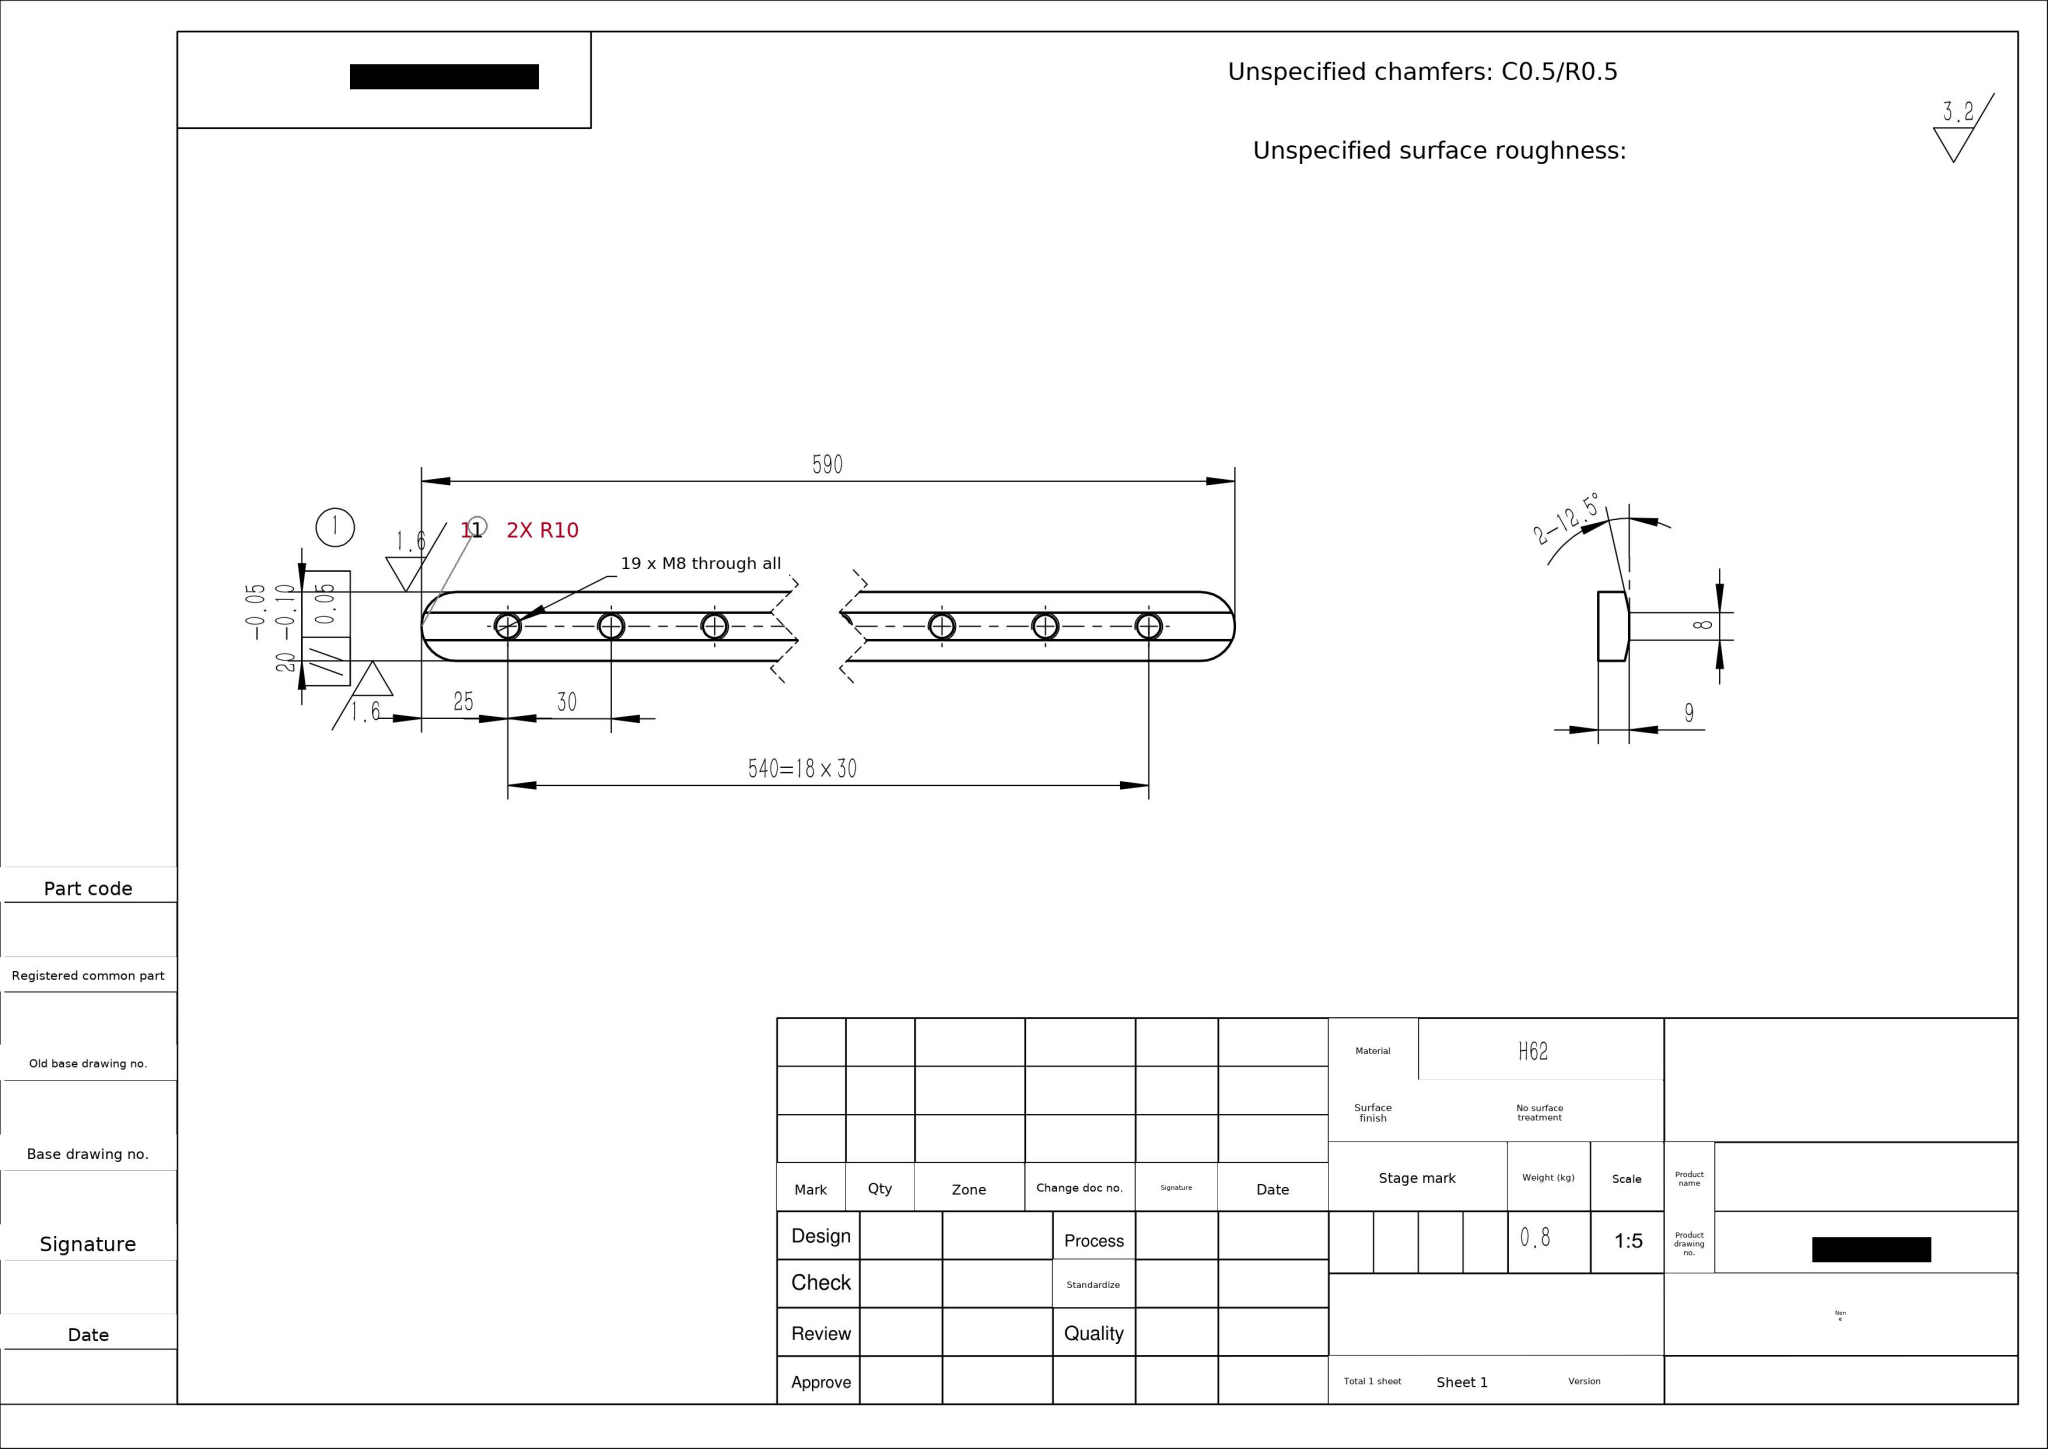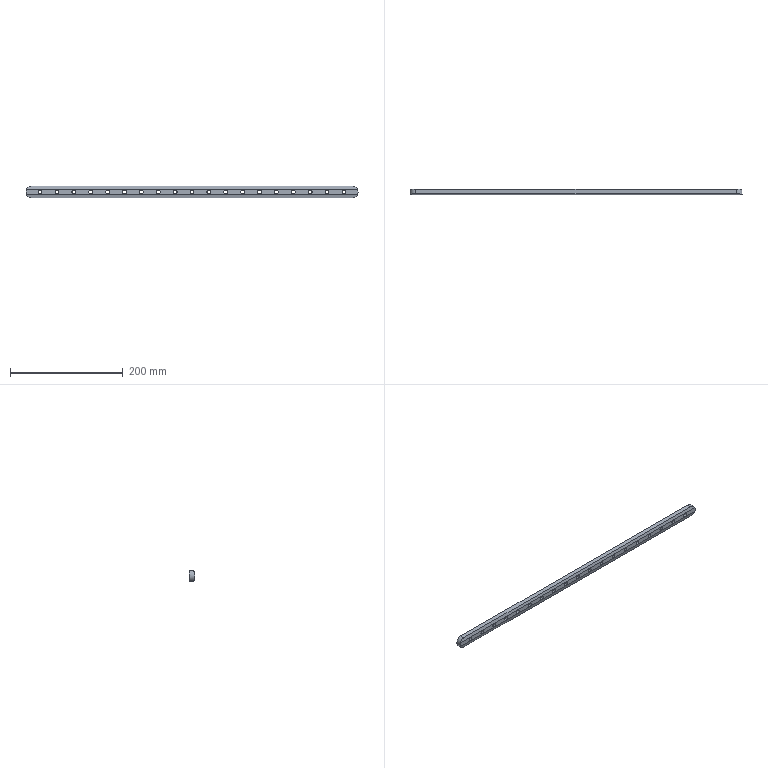Part | SolidWorks | mm | material H62 | 1 solid | 46 faces | box 590 x 9 x 20 mm | volume 94581 mm3 | cylinder 40 | plane 6 | commonest cylinder face diameters 6.8 x38 20 x2
build123d program:
from build123d import *

# Parameters (mm, degrees)
BOSS_EXTRUDE1_DEPTH = 9
M8_TAPPED_HOLE1_D   = 6.8
LPATTERN1_COUNT     = 19
LPATTERN1_PITCH     = 30
CUT_EXTRUDE1_START  = -200
CUT_EXTRUDE1_DEPTH  = 690.208


with BuildPart() as part:
    # Sketch1 → Boss-Extrude1 (new body)
    with BuildSketch(Plane(origin=(0, 0, 0), x_dir=(1, 0, 0), z_dir=(0, 1, 0))):
        with BuildLine():
            Line((-90.977, 10), (479.023, 10))
            ThreePointArc((479.023, 10), (489.023, 0), (479.023, -10))
            Line((479.023, -10), (-90.977, -10))
            ThreePointArc((-90.977, -10), (-100.977, 0), (-90.977, 10))
        make_face()
    extrude(amount=BOSS_EXTRUDE1_DEPTH)

    # M8 Tapped Hole1 (through all)
    with Locations(Plane(origin=(0, 9, 0), x_dir=(1, 0, 0), z_dir=(0, 1, 0))):
        with Locations((-75.977, 0)):
            m8_tapped_hole1 = Hole(M8_TAPPED_HOLE1_D / 2)

    # LPattern1: M8 Tapped Hole1 ×19
    with Locations(*[(i * LPATTERN1_PITCH, 0, 0) for i in range(1, LPATTERN1_COUNT)]):
        add(m8_tapped_hole1, mode=Mode.SUBTRACT)

    # Sketch4 → Cut-Extrude1 (cut, through all)
    with BuildSketch(Plane(origin=(0, 0, 0), x_dir=(0, 0, -1), z_dir=(1, 0, 0)).offset(CUT_EXTRUDE1_START)):
        Polygon((4, 0), (14, 0), (14, 2.217), align=None)
        Polygon((-14, 2.217), (-14, 0), (-4, 0), align=None)
    extrude(amount=CUT_EXTRUDE1_DEPTH, mode=Mode.SUBTRACT)


solid = part.part